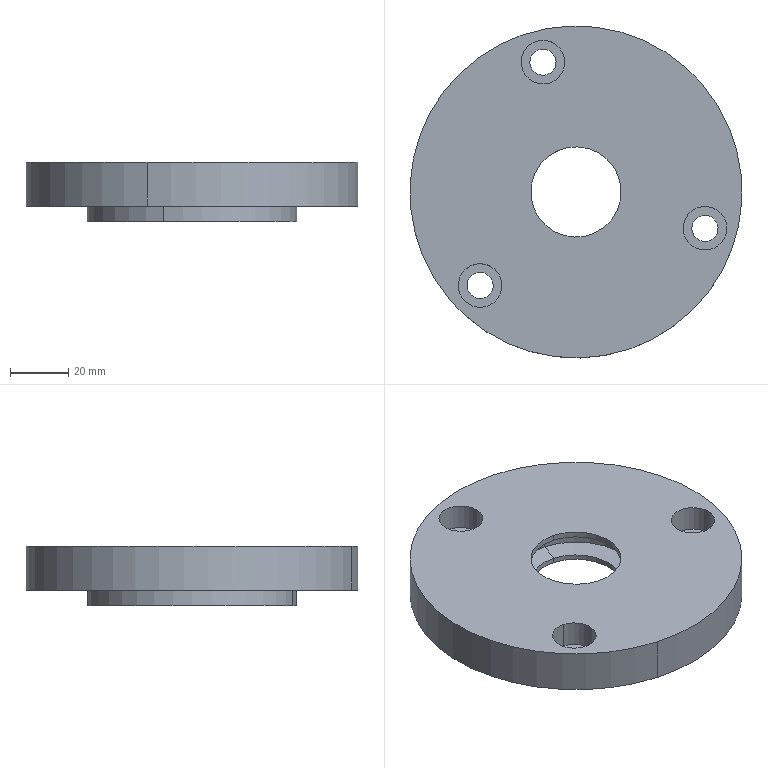Component | SolidWorks | 227-2 | 1 solid | 37 faces | box 114 x 114 x 20.3 mm | volume 130185 mm3 | cylinder 24 | plane 7 | cone 4 | torus 2 | commonest cylinder face diameters 15 x6 9 x6 31 x4 44 x2 60 x2 72 x2 114 x2
STEP:
#1=COLOUR_RGB('',0.7922,0.8196,0.9333);
#2=FILL_AREA_STYLE_COLOUR('',#1);
#3=FILL_AREA_STYLE('',(#2));
#4=SURFACE_STYLE_FILL_AREA(#3);
#5=SURFACE_SIDE_STYLE('',(#4));
#6=SURFACE_STYLE_USAGE(.BOTH.,#5);
#7=PRESENTATION_STYLE_ASSIGNMENT((#6));
#8=CARTESIAN_POINT('',(3.044,-0.8272,3.035));
#9=VERTEX_POINT('',#8);
#10=CARTESIAN_POINT('',(2.468,-2.874,3.035));
#11=VERTEX_POINT('',#10);
#12=CARTESIAN_POINT('',(2.756,-1.85,3.035));
#13=DIRECTION('',(0.,-0.,-1.));
#14=DIRECTION('',(-0.271,-0.9626,0.));
#15=AXIS2_PLACEMENT_3D('',#12,#13,#14);
#16=CIRCLE('',#15,1.063);
#17=EDGE_CURVE('',#9,#11,#16,.T.);
#18=ORIENTED_EDGE('',*,*,#17,.F.);
#19=CARTESIAN_POINT('',(3.076,-0.7135,2.917));
#20=VERTEX_POINT('',#19);
#21=CARTESIAN_POINT('',(3.044,-0.8272,2.917));
#22=DIRECTION('',(-0.9626,0.271,-0.));
#23=DIRECTION('',(-0.271,-0.9626,0.));
#24=AXIS2_PLACEMENT_3D('',#21,#22,#23);
#25=CIRCLE('',#24,0.1181);
#26=EDGE_CURVE('',#9,#20,#25,.T.);
#27=ORIENTED_EDGE('',*,*,#26,.T.);
#28=CARTESIAN_POINT('',(2.436,-2.987,2.917));
#29=VERTEX_POINT('',#28);
#30=CARTESIAN_POINT('',(2.756,-1.85,2.917));
#31=DIRECTION('',(-0.,0.,1.));
#32=DIRECTION('',(-0.271,-0.9626,0.));
#33=AXIS2_PLACEMENT_3D('',#30,#31,#32);
#34=CIRCLE('',#33,1.181);
#35=EDGE_CURVE('',#29,#20,#34,.T.);
#36=ORIENTED_EDGE('',*,*,#35,.F.);
#37=CARTESIAN_POINT('',(2.468,-2.874,2.917));
#38=DIRECTION('',(0.9626,-0.271,0.));
#39=DIRECTION('',(0.271,0.9626,0.));
#40=AXIS2_PLACEMENT_3D('',#37,#38,#39);
#41=CIRCLE('',#40,0.1181);
#42=EDGE_CURVE('',#11,#29,#41,.T.);
#43=ORIENTED_EDGE('',*,*,#42,.F.);
#44=EDGE_LOOP('',(#18,#27,#36,#43));
#45=FACE_OUTER_BOUND('',#44,.T.);
#46=CARTESIAN_POINT('',(2.756,-1.85,2.917));
#47=DIRECTION('',(0.,-0.,-1.));
#48=DIRECTION('',(-0.271,-0.9626,0.));
#49=AXIS2_PLACEMENT_3D('',#46,#47,#48);
#50=TOROIDAL_SURFACE('',#49,1.063,0.1181);
#51=ADVANCED_FACE('',(#45),#50,.F.);
#52=CARTESIAN_POINT('',(4.785,-2.268,3.13));
#53=VERTEX_POINT('',#52);
#54=CARTESIAN_POINT('',(4.213,-2.414,3.13));
#55=VERTEX_POINT('',#54);
#56=CARTESIAN_POINT('',(4.499,-2.341,3.13));
#57=DIRECTION('',(-0.,0.,1.));
#58=DIRECTION('',(-0.9691,-0.2466,0.));
#59=AXIS2_PLACEMENT_3D('',#56,#57,#58);
#60=CIRCLE('',#59,0.2953);
#61=EDGE_CURVE('',#53,#55,#60,.T.);
#62=ORIENTED_EDGE('',*,*,#61,.F.);
#63=CARTESIAN_POINT('',(4.785,-2.268,3.484));
#64=VERTEX_POINT('',#63);
#65=CARTESIAN_POINT('',(4.785,-2.268,3.13));
#66=DIRECTION('',(-0.,0.,1.));
#67=VECTOR('',#66,39.37);
#68=LINE('',#65,#67);
#69=EDGE_CURVE('',#53,#64,#68,.T.);
#70=ORIENTED_EDGE('',*,*,#69,.T.);
#71=CARTESIAN_POINT('',(4.213,-2.414,3.484));
#72=VERTEX_POINT('',#71);
#73=CARTESIAN_POINT('',(4.499,-2.341,3.484));
#74=DIRECTION('',(-0.,0.,1.));
#75=DIRECTION('',(-0.9691,-0.2466,0.));
#76=AXIS2_PLACEMENT_3D('',#73,#74,#75);
#77=CIRCLE('',#76,0.2953);
#78=EDGE_CURVE('',#64,#72,#77,.T.);
#79=ORIENTED_EDGE('',*,*,#78,.T.);
#80=CARTESIAN_POINT('',(4.213,-2.414,3.13));
#81=DIRECTION('',(-0.,0.,1.));
#82=VECTOR('',#81,39.37);
#83=LINE('',#80,#82);
#84=EDGE_CURVE('',#55,#72,#83,.T.);
#85=ORIENTED_EDGE('',*,*,#84,.F.);
#86=EDGE_LOOP('',(#62,#70,#79,#85));
#87=FACE_OUTER_BOUND('',#86,.T.);
#88=CARTESIAN_POINT('',(4.499,-2.341,3.13));
#89=DIRECTION('',(-0.,0.,1.));
#90=DIRECTION('',(-0.9691,-0.2466,0.));
#91=AXIS2_PLACEMENT_3D('',#88,#89,#90);
#92=CYLINDRICAL_SURFACE('',#91,0.2953);
#93=ADVANCED_FACE('',(#87),#92,.F.);
#94=CARTESIAN_POINT('',(2.103,0.1161,3.13));
#95=VERTEX_POINT('',#94);
#96=CARTESIAN_POINT('',(2.515,-0.3067,3.13));
#97=VERTEX_POINT('',#96);
#98=CARTESIAN_POINT('',(2.309,-0.09529,3.13));
#99=DIRECTION('',(-0.,0.,1.));
#100=DIRECTION('',(0.6981,-0.716,0.));
#101=AXIS2_PLACEMENT_3D('',#98,#99,#100);
#102=CIRCLE('',#101,0.2953);
#103=EDGE_CURVE('',#95,#97,#102,.T.);
#104=ORIENTED_EDGE('',*,*,#103,.F.);
#105=CARTESIAN_POINT('',(2.103,0.1161,3.484));
#106=VERTEX_POINT('',#105);
#107=CARTESIAN_POINT('',(2.103,0.1161,3.13));
#108=DIRECTION('',(-0.,0.,1.));
#109=VECTOR('',#108,39.37);
#110=LINE('',#107,#109);
#111=EDGE_CURVE('',#95,#106,#110,.T.);
#112=ORIENTED_EDGE('',*,*,#111,.T.);
#113=CARTESIAN_POINT('',(2.515,-0.3067,3.484));
#114=VERTEX_POINT('',#113);
#115=CARTESIAN_POINT('',(2.309,-0.09529,3.484));
#116=DIRECTION('',(-0.,0.,1.));
#117=DIRECTION('',(0.6981,-0.716,0.));
#118=AXIS2_PLACEMENT_3D('',#115,#116,#117);
#119=CIRCLE('',#118,0.2953);
#120=EDGE_CURVE('',#106,#114,#119,.T.);
#121=ORIENTED_EDGE('',*,*,#120,.T.);
#122=CARTESIAN_POINT('',(2.515,-0.3067,3.13));
#123=DIRECTION('',(-0.,0.,1.));
#124=VECTOR('',#123,39.37);
#125=LINE('',#122,#124);
#126=EDGE_CURVE('',#97,#114,#125,.T.);
#127=ORIENTED_EDGE('',*,*,#126,.F.);
#128=EDGE_LOOP('',(#104,#112,#121,#127));
#129=FACE_OUTER_BOUND('',#128,.T.);
#130=CARTESIAN_POINT('',(2.309,-0.09529,3.13));
#131=DIRECTION('',(-0.,0.,1.));
#132=DIRECTION('',(0.6981,-0.716,0.));
#133=AXIS2_PLACEMENT_3D('',#130,#131,#132);
#134=CYLINDRICAL_SURFACE('',#133,0.2953);
#135=ADVANCED_FACE('',(#129),#134,.F.);
#136=CARTESIAN_POINT('',(1.379,-3.399,3.13));
#137=VERTEX_POINT('',#136);
#138=CARTESIAN_POINT('',(1.539,-2.83,3.13));
#139=VERTEX_POINT('',#138);
#140=CARTESIAN_POINT('',(1.459,-3.115,3.13));
#141=DIRECTION('',(-0.,0.,1.));
#142=DIRECTION('',(0.271,0.9626,0.));
#143=AXIS2_PLACEMENT_3D('',#140,#141,#142);
#144=CIRCLE('',#143,0.2953);
#145=EDGE_CURVE('',#137,#139,#144,.T.);
#146=ORIENTED_EDGE('',*,*,#145,.F.);
#147=CARTESIAN_POINT('',(1.379,-3.399,3.484));
#148=VERTEX_POINT('',#147);
#149=CARTESIAN_POINT('',(1.379,-3.399,3.13));
#150=DIRECTION('',(-0.,0.,1.));
#151=VECTOR('',#150,39.37);
#152=LINE('',#149,#151);
#153=EDGE_CURVE('',#137,#148,#152,.T.);
#154=ORIENTED_EDGE('',*,*,#153,.T.);
#155=CARTESIAN_POINT('',(1.539,-2.83,3.484));
#156=VERTEX_POINT('',#155);
#157=CARTESIAN_POINT('',(1.459,-3.115,3.484));
#158=DIRECTION('',(-0.,0.,1.));
#159=DIRECTION('',(0.271,0.9626,0.));
#160=AXIS2_PLACEMENT_3D('',#157,#158,#159);
#161=CIRCLE('',#160,0.2953);
#162=EDGE_CURVE('',#148,#156,#161,.T.);
#163=ORIENTED_EDGE('',*,*,#162,.T.);
#164=CARTESIAN_POINT('',(1.539,-2.83,3.13));
#165=DIRECTION('',(-0.,0.,1.));
#166=VECTOR('',#165,39.37);
#167=LINE('',#164,#166);
#168=EDGE_CURVE('',#139,#156,#167,.T.);
#169=ORIENTED_EDGE('',*,*,#168,.F.);
#170=EDGE_LOOP('',(#146,#154,#163,#169));
#171=FACE_OUTER_BOUND('',#170,.T.);
#172=CARTESIAN_POINT('',(1.459,-3.115,3.13));
#173=DIRECTION('',(-0.,0.,1.));
#174=DIRECTION('',(0.271,0.9626,0.));
#175=AXIS2_PLACEMENT_3D('',#172,#173,#174);
#176=CYLINDRICAL_SURFACE('',#175,0.2953);
#177=ADVANCED_FACE('',(#171),#176,.F.);
#178=CARTESIAN_POINT('',(2.921,-1.263,3.106));
#179=VERTEX_POINT('',#178);
#180=CARTESIAN_POINT('',(2.591,-2.438,3.106));
#181=VERTEX_POINT('',#180);
#182=CARTESIAN_POINT('',(2.756,-1.85,3.106));
#183=DIRECTION('',(0.,-0.,-1.));
#184=DIRECTION('',(-0.271,-0.9626,0.));
#185=AXIS2_PLACEMENT_3D('',#182,#183,#184);
#186=CIRCLE('',#185,0.6102);
#187=EDGE_CURVE('',#179,#181,#186,.T.);
#188=ORIENTED_EDGE('',*,*,#187,.F.);
#189=CARTESIAN_POINT('',(2.921,-1.263,3.035));
#190=VERTEX_POINT('',#189);
#191=CARTESIAN_POINT('',(2.921,-1.263,2.783));
#192=DIRECTION('',(0.,-0.,-1.));
#193=VECTOR('',#192,39.37);
#194=LINE('',#191,#193);
#195=EDGE_CURVE('',#179,#190,#194,.T.);
#196=ORIENTED_EDGE('',*,*,#195,.T.);
#197=CARTESIAN_POINT('',(2.591,-2.438,3.035));
#198=VERTEX_POINT('',#197);
#199=CARTESIAN_POINT('',(2.756,-1.85,3.035));
#200=DIRECTION('',(0.,-0.,-1.));
#201=DIRECTION('',(-0.271,-0.9626,0.));
#202=AXIS2_PLACEMENT_3D('',#199,#200,#201);
#203=CIRCLE('',#202,0.6102);
#204=EDGE_CURVE('',#190,#198,#203,.T.);
#205=ORIENTED_EDGE('',*,*,#204,.T.);
#206=CARTESIAN_POINT('',(2.591,-2.438,2.783));
#207=DIRECTION('',(0.,-0.,-1.));
#208=VECTOR('',#207,39.37);
#209=LINE('',#206,#208);
#210=EDGE_CURVE('',#181,#198,#209,.T.);
#211=ORIENTED_EDGE('',*,*,#210,.F.);
#212=EDGE_LOOP('',(#188,#196,#205,#211));
#213=FACE_OUTER_BOUND('',#212,.T.);
#214=CARTESIAN_POINT('',(2.756,-1.85,2.783));
#215=DIRECTION('',(0.,-0.,-1.));
#216=DIRECTION('',(-0.271,-0.9626,0.));
#217=AXIS2_PLACEMENT_3D('',#214,#215,#216);
#218=CYLINDRICAL_SURFACE('',#217,0.6102);
#219=ADVANCED_FACE('',(#213),#218,.F.);
#220=ORIENTED_EDGE('',*,*,#187,.T.);
#221=CARTESIAN_POINT('',(2.521,-2.684,3.138));
#222=VERTEX_POINT('',#221);
#223=CARTESIAN_POINT('',(2.591,-2.438,3.106));
#224=DIRECTION('',(-0.269,-0.9554,0.1219));
#225=VECTOR('',#224,39.37);
#226=LINE('',#223,#225);
#227=EDGE_CURVE('',#181,#222,#226,.T.);
#228=ORIENTED_EDGE('',*,*,#227,.T.);
#229=CARTESIAN_POINT('',(2.991,-1.017,3.138));
#230=VERTEX_POINT('',#229);
#231=CARTESIAN_POINT('',(2.756,-1.85,3.138));
#232=DIRECTION('',(0.,-0.,-1.));
#233=DIRECTION('',(-0.271,-0.9626,0.));
#234=AXIS2_PLACEMENT_3D('',#231,#232,#233);
#235=CIRCLE('',#234,0.8661);
#236=EDGE_CURVE('',#230,#222,#235,.T.);
#237=ORIENTED_EDGE('',*,*,#236,.F.);
#238=CARTESIAN_POINT('',(2.921,-1.263,3.106));
#239=DIRECTION('',(0.269,0.9554,0.1219));
#240=VECTOR('',#239,39.37);
#241=LINE('',#238,#240);
#242=EDGE_CURVE('',#179,#230,#241,.T.);
#243=ORIENTED_EDGE('',*,*,#242,.F.);
#244=EDGE_LOOP('',(#220,#228,#237,#243));
#245=FACE_OUTER_BOUND('',#244,.T.);
#246=CARTESIAN_POINT('',(2.756,-1.85,3.106));
#247=DIRECTION('',(-0.,0.,1.));
#248=DIRECTION('',(0.271,0.9626,0.));
#249=AXIS2_PLACEMENT_3D('',#246,#247,#248);
#250=CONICAL_SURFACE('',#249,0.6102,1.449);
#251=ADVANCED_FACE('',(#245),#250,.F.);
#252=CARTESIAN_POINT('',(2.991,-1.017,3.374));
#253=VERTEX_POINT('',#252);
#254=CARTESIAN_POINT('',(2.521,-2.684,3.374));
#255=VERTEX_POINT('',#254);
#256=CARTESIAN_POINT('',(2.756,-1.85,3.374));
#257=DIRECTION('',(0.,-0.,-1.));
#258=DIRECTION('',(-0.271,-0.9626,0.));
#259=AXIS2_PLACEMENT_3D('',#256,#257,#258);
#260=CIRCLE('',#259,0.8661);
#261=EDGE_CURVE('',#253,#255,#260,.T.);
#262=ORIENTED_EDGE('',*,*,#261,.F.);
#263=CARTESIAN_POINT('',(2.991,-1.017,2.783));
#264=DIRECTION('',(0.,-0.,-1.));
#265=VECTOR('',#264,39.37);
#266=LINE('',#263,#265);
#267=EDGE_CURVE('',#253,#230,#266,.T.);
#268=ORIENTED_EDGE('',*,*,#267,.T.);
#269=ORIENTED_EDGE('',*,*,#236,.T.);
#270=CARTESIAN_POINT('',(2.521,-2.684,2.783));
#271=DIRECTION('',(0.,-0.,-1.));
#272=VECTOR('',#271,39.37);
#273=LINE('',#270,#272);
#274=EDGE_CURVE('',#255,#222,#273,.T.);
#275=ORIENTED_EDGE('',*,*,#274,.F.);
#276=EDGE_LOOP('',(#262,#268,#269,#275));
#277=FACE_OUTER_BOUND('',#276,.T.);
#278=CARTESIAN_POINT('',(2.756,-1.85,2.783));
#279=DIRECTION('',(0.,-0.,-1.));
#280=DIRECTION('',(-0.271,-0.9626,0.));
#281=AXIS2_PLACEMENT_3D('',#278,#279,#280);
#282=CYLINDRICAL_SURFACE('',#281,0.8661);
#283=ADVANCED_FACE('',(#277),#282,.F.);
#284=CARTESIAN_POINT('',(2.921,-1.263,3.405));
#285=VERTEX_POINT('',#284);
#286=CARTESIAN_POINT('',(2.591,-2.438,3.405));
#287=VERTEX_POINT('',#286);
#288=CARTESIAN_POINT('',(2.756,-1.85,3.405));
#289=DIRECTION('',(0.,-0.,-1.));
#290=DIRECTION('',(-0.271,-0.9626,0.));
#291=AXIS2_PLACEMENT_3D('',#288,#289,#290);
#292=CIRCLE('',#291,0.6102);
#293=EDGE_CURVE('',#285,#287,#292,.T.);
#294=ORIENTED_EDGE('',*,*,#293,.F.);
#295=CARTESIAN_POINT('',(2.991,-1.017,3.374));
#296=DIRECTION('',(0.269,0.9554,-0.1219));
#297=VECTOR('',#296,39.37);
#298=LINE('',#295,#297);
#299=EDGE_CURVE('',#285,#253,#298,.T.);
#300=ORIENTED_EDGE('',*,*,#299,.T.);
#301=ORIENTED_EDGE('',*,*,#261,.T.);
#302=CARTESIAN_POINT('',(2.521,-2.684,3.374));
#303=DIRECTION('',(-0.269,-0.9554,-0.1219));
#304=VECTOR('',#303,39.37);
#305=LINE('',#302,#304);
#306=EDGE_CURVE('',#287,#255,#305,.T.);
#307=ORIENTED_EDGE('',*,*,#306,.F.);
#308=EDGE_LOOP('',(#294,#300,#301,#307));
#309=FACE_OUTER_BOUND('',#308,.T.);
#310=CARTESIAN_POINT('',(2.756,-1.85,3.374));
#311=DIRECTION('',(0.,-0.,-1.));
#312=DIRECTION('',(-0.271,-0.9626,0.));
#313=AXIS2_PLACEMENT_3D('',#310,#311,#312);
#314=CONICAL_SURFACE('',#313,0.8661,1.449);
#315=ADVANCED_FACE('',(#309),#314,.F.);
#316=CARTESIAN_POINT('',(2.921,-1.263,3.484));
#317=VERTEX_POINT('',#316);
#318=CARTESIAN_POINT('',(2.591,-2.438,3.484));
#319=VERTEX_POINT('',#318);
#320=CARTESIAN_POINT('',(2.756,-1.85,3.484));
#321=DIRECTION('',(0.,-0.,-1.));
#322=DIRECTION('',(-0.271,-0.9626,0.));
#323=AXIS2_PLACEMENT_3D('',#320,#321,#322);
#324=CIRCLE('',#323,0.6102);
#325=EDGE_CURVE('',#317,#319,#324,.T.);
#326=ORIENTED_EDGE('',*,*,#325,.F.);
#327=CARTESIAN_POINT('',(2.921,-1.263,2.783));
#328=DIRECTION('',(0.,-0.,-1.));
#329=VECTOR('',#328,39.37);
#330=LINE('',#327,#329);
#331=EDGE_CURVE('',#317,#285,#330,.T.);
#332=ORIENTED_EDGE('',*,*,#331,.T.);
#333=ORIENTED_EDGE('',*,*,#293,.T.);
#334=CARTESIAN_POINT('',(2.591,-2.438,2.783));
#335=DIRECTION('',(0.,-0.,-1.));
#336=VECTOR('',#335,39.37);
#337=LINE('',#334,#336);
#338=EDGE_CURVE('',#319,#287,#337,.T.);
#339=ORIENTED_EDGE('',*,*,#338,.F.);
#340=EDGE_LOOP('',(#326,#332,#333,#339));
#341=FACE_OUTER_BOUND('',#340,.T.);
#342=CARTESIAN_POINT('',(2.756,-1.85,2.783));
#343=DIRECTION('',(0.,-0.,-1.));
#344=DIRECTION('',(-0.271,-0.9626,0.));
#345=AXIS2_PLACEMENT_3D('',#342,#343,#344);
#346=CYLINDRICAL_SURFACE('',#345,0.6102);
#347=ADVANCED_FACE('',(#341),#346,.F.);
#348=ORIENTED_EDGE('',*,*,#35,.T.);
#349=CARTESIAN_POINT('',(3.076,-0.7135,2.685));
#350=VERTEX_POINT('',#349);
#351=CARTESIAN_POINT('',(3.076,-0.7135,6.825));
#352=DIRECTION('',(0.,-0.,-1.));
#353=VECTOR('',#352,39.37);
#354=LINE('',#351,#353);
#355=EDGE_CURVE('',#20,#350,#354,.T.);
#356=ORIENTED_EDGE('',*,*,#355,.T.);
#357=CARTESIAN_POINT('',(2.436,-2.987,2.685));
#358=VERTEX_POINT('',#357);
#359=CARTESIAN_POINT('',(2.756,-1.85,2.685));
#360=DIRECTION('',(0.,-0.,-1.));
#361=DIRECTION('',(-0.271,-0.9626,0.));
#362=AXIS2_PLACEMENT_3D('',#359,#360,#361);
#363=CIRCLE('',#362,1.181);
#364=EDGE_CURVE('',#350,#358,#363,.T.);
#365=ORIENTED_EDGE('',*,*,#364,.T.);
#366=CARTESIAN_POINT('',(2.436,-2.987,6.825));
#367=DIRECTION('',(0.,-0.,-1.));
#368=VECTOR('',#367,39.37);
#369=LINE('',#366,#368);
#370=EDGE_CURVE('',#29,#358,#369,.T.);
#371=ORIENTED_EDGE('',*,*,#370,.F.);
#372=EDGE_LOOP('',(#348,#356,#365,#371));
#373=FACE_OUTER_BOUND('',#372,.T.);
#374=CARTESIAN_POINT('',(2.756,-1.85,6.825));
#375=DIRECTION('',(0.,-0.,-1.));
#376=DIRECTION('',(-0.271,-0.9626,0.));
#377=AXIS2_PLACEMENT_3D('',#374,#375,#376);
#378=CYLINDRICAL_SURFACE('',#377,1.181);
#379=ADVANCED_FACE('',(#373),#378,.F.);
#380=CARTESIAN_POINT('',(2.372,-3.215,2.685));
#381=VERTEX_POINT('',#380);
#382=CARTESIAN_POINT('',(3.14,-0.4861,2.685));
#383=VERTEX_POINT('',#382);
#384=CARTESIAN_POINT('',(2.756,-1.85,2.685));
#385=DIRECTION('',(0.,-0.,-1.));
#386=DIRECTION('',(-0.271,-0.9626,0.));
#387=AXIS2_PLACEMENT_3D('',#384,#385,#386);
#388=CIRCLE('',#387,1.417);
#389=EDGE_CURVE('',#381,#383,#388,.T.);
#390=ORIENTED_EDGE('',*,*,#389,.F.);
#391=CARTESIAN_POINT('',(2.372,-3.215,2.894));
#392=VERTEX_POINT('',#391);
#393=CARTESIAN_POINT('',(2.372,-3.215,2.685));
#394=DIRECTION('',(-0.,0.,1.));
#395=VECTOR('',#394,39.37);
#396=LINE('',#393,#395);
#397=EDGE_CURVE('',#381,#392,#396,.T.);
#398=ORIENTED_EDGE('',*,*,#397,.T.);
#399=CARTESIAN_POINT('',(3.14,-0.4861,2.894));
#400=VERTEX_POINT('',#399);
#401=CARTESIAN_POINT('',(2.756,-1.85,2.894));
#402=DIRECTION('',(0.,-0.,-1.));
#403=DIRECTION('',(-0.271,-0.9626,0.));
#404=AXIS2_PLACEMENT_3D('',#401,#402,#403);
#405=CIRCLE('',#404,1.417);
#406=EDGE_CURVE('',#392,#400,#405,.T.);
#407=ORIENTED_EDGE('',*,*,#406,.T.);
#408=CARTESIAN_POINT('',(3.14,-0.4861,2.685));
#409=DIRECTION('',(-0.,0.,1.));
#410=VECTOR('',#409,39.37);
#411=LINE('',#408,#410);
#412=EDGE_CURVE('',#383,#400,#411,.T.);
#413=ORIENTED_EDGE('',*,*,#412,.F.);
#414=EDGE_LOOP('',(#390,#398,#407,#413));
#415=FACE_OUTER_BOUND('',#414,.T.);
#416=CARTESIAN_POINT('',(2.756,-1.85,2.685));
#417=DIRECTION('',(-0.,0.,1.));
#418=DIRECTION('',(0.271,0.9626,0.));
#419=AXIS2_PLACEMENT_3D('',#416,#417,#418);
#420=CYLINDRICAL_SURFACE('',#419,1.417);
#421=ADVANCED_FACE('',(#415),#420,.T.);
#422=CARTESIAN_POINT('',(2.148,-4.011,2.894));
#423=VERTEX_POINT('',#422);
#424=CARTESIAN_POINT('',(3.364,0.3097,2.894));
#425=VERTEX_POINT('',#424);
#426=CARTESIAN_POINT('',(2.756,-1.85,2.894));
#427=DIRECTION('',(0.,-0.,-1.));
#428=DIRECTION('',(-0.271,-0.9626,0.));
#429=AXIS2_PLACEMENT_3D('',#426,#427,#428);
#430=CIRCLE('',#429,2.244);
#431=EDGE_CURVE('',#423,#425,#430,.T.);
#432=ORIENTED_EDGE('',*,*,#431,.F.);
#433=CARTESIAN_POINT('',(2.148,-4.011,3.484));
#434=VERTEX_POINT('',#433);
#435=CARTESIAN_POINT('',(2.148,-4.011,2.894));
#436=DIRECTION('',(-0.,0.,1.));
#437=VECTOR('',#436,39.37);
#438=LINE('',#435,#437);
#439=EDGE_CURVE('',#423,#434,#438,.T.);
#440=ORIENTED_EDGE('',*,*,#439,.T.);
#441=CARTESIAN_POINT('',(3.364,0.3097,3.484));
#442=VERTEX_POINT('',#441);
#443=CARTESIAN_POINT('',(2.756,-1.85,3.484));
#444=DIRECTION('',(0.,-0.,-1.));
#445=DIRECTION('',(-0.271,-0.9626,0.));
#446=AXIS2_PLACEMENT_3D('',#443,#444,#445);
#447=CIRCLE('',#446,2.244);
#448=EDGE_CURVE('',#434,#442,#447,.T.);
#449=ORIENTED_EDGE('',*,*,#448,.T.);
#450=CARTESIAN_POINT('',(3.364,0.3097,2.894));
#451=DIRECTION('',(-0.,0.,1.));
#452=VECTOR('',#451,39.37);
#453=LINE('',#450,#452);
#454=EDGE_CURVE('',#425,#442,#453,.T.);
#455=ORIENTED_EDGE('',*,*,#454,.F.);
#456=EDGE_LOOP('',(#432,#440,#449,#455));
#457=FACE_OUTER_BOUND('',#456,.T.);
#458=CARTESIAN_POINT('',(2.756,-1.85,2.894));
#459=DIRECTION('',(-0.,0.,1.));
#460=DIRECTION('',(0.271,0.9626,0.));
#461=AXIS2_PLACEMENT_3D('',#458,#459,#460);
#462=CYLINDRICAL_SURFACE('',#461,2.244);
#463=ADVANCED_FACE('',(#457),#462,.T.);
#464=CARTESIAN_POINT('',(1.507,-2.944,2.894));
#465=VERTEX_POINT('',#464);
#466=CARTESIAN_POINT('',(1.411,-3.285,2.894));
#467=VERTEX_POINT('',#466);
#468=CARTESIAN_POINT('',(1.459,-3.115,2.894));
#469=DIRECTION('',(0.,-0.,-1.));
#470=DIRECTION('',(-0.271,-0.9626,0.));
#471=AXIS2_PLACEMENT_3D('',#468,#469,#470);
#472=CIRCLE('',#471,0.1772);
#473=EDGE_CURVE('',#465,#467,#472,.T.);
#474=ORIENTED_EDGE('',*,*,#473,.T.);
#475=CARTESIAN_POINT('',(1.411,-3.285,3.13));
#476=VERTEX_POINT('',#475);
#477=CARTESIAN_POINT('',(1.411,-3.285,2.894));
#478=DIRECTION('',(-0.,0.,1.));
#479=VECTOR('',#478,39.37);
#480=LINE('',#477,#479);
#481=EDGE_CURVE('',#467,#476,#480,.T.);
#482=ORIENTED_EDGE('',*,*,#481,.T.);
#483=CARTESIAN_POINT('',(1.507,-2.944,3.13));
#484=VERTEX_POINT('',#483);
#485=CARTESIAN_POINT('',(1.459,-3.115,3.13));
#486=DIRECTION('',(-0.,0.,1.));
#487=DIRECTION('',(0.271,0.9626,0.));
#488=AXIS2_PLACEMENT_3D('',#485,#486,#487);
#489=CIRCLE('',#488,0.1772);
#490=EDGE_CURVE('',#476,#484,#489,.T.);
#491=ORIENTED_EDGE('',*,*,#490,.T.);
#492=CARTESIAN_POINT('',(1.507,-2.944,2.894));
#493=DIRECTION('',(-0.,0.,1.));
#494=VECTOR('',#493,39.37);
#495=LINE('',#492,#494);
#496=EDGE_CURVE('',#465,#484,#495,.T.);
#497=ORIENTED_EDGE('',*,*,#496,.F.);
#498=EDGE_LOOP('',(#474,#482,#491,#497));
#499=FACE_OUTER_BOUND('',#498,.T.);
#500=CARTESIAN_POINT('',(1.459,-3.115,2.894));
#501=DIRECTION('',(-0.,0.,1.));
#502=DIRECTION('',(0.271,0.9626,0.));
#503=AXIS2_PLACEMENT_3D('',#500,#501,#502);
#504=CYLINDRICAL_SURFACE('',#503,0.1772);
#505=ADVANCED_FACE('',(#499),#504,.F.);
#506=CARTESIAN_POINT('',(2.357,0.07525,2.894));
#507=VERTEX_POINT('',#506);
#508=CARTESIAN_POINT('',(2.261,-0.2658,2.894));
#509=VERTEX_POINT('',#508);
#510=CARTESIAN_POINT('',(2.309,-0.09529,2.894));
#511=DIRECTION('',(0.,-0.,-1.));
#512=DIRECTION('',(-0.271,-0.9626,0.));
#513=AXIS2_PLACEMENT_3D('',#510,#511,#512);
#514=CIRCLE('',#513,0.1772);
#515=EDGE_CURVE('',#507,#509,#514,.T.);
#516=ORIENTED_EDGE('',*,*,#515,.T.);
#517=CARTESIAN_POINT('',(2.261,-0.2658,3.13));
#518=VERTEX_POINT('',#517);
#519=CARTESIAN_POINT('',(2.261,-0.2658,2.894));
#520=DIRECTION('',(-0.,0.,1.));
#521=VECTOR('',#520,39.37);
#522=LINE('',#519,#521);
#523=EDGE_CURVE('',#509,#518,#522,.T.);
#524=ORIENTED_EDGE('',*,*,#523,.T.);
#525=CARTESIAN_POINT('',(2.357,0.07525,3.13));
#526=VERTEX_POINT('',#525);
#527=CARTESIAN_POINT('',(2.309,-0.09529,3.13));
#528=DIRECTION('',(-0.,0.,1.));
#529=DIRECTION('',(0.271,0.9626,0.));
#530=AXIS2_PLACEMENT_3D('',#527,#528,#529);
#531=CIRCLE('',#530,0.1772);
#532=EDGE_CURVE('',#518,#526,#531,.T.);
#533=ORIENTED_EDGE('',*,*,#532,.T.);
#534=CARTESIAN_POINT('',(2.357,0.07525,2.894));
#535=DIRECTION('',(-0.,0.,1.));
#536=VECTOR('',#535,39.37);
#537=LINE('',#534,#536);
#538=EDGE_CURVE('',#507,#526,#537,.T.);
#539=ORIENTED_EDGE('',*,*,#538,.F.);
#540=EDGE_LOOP('',(#516,#524,#533,#539));
#541=FACE_OUTER_BOUND('',#540,.T.);
#542=CARTESIAN_POINT('',(2.309,-0.09529,2.894));
#543=DIRECTION('',(-0.,0.,1.));
#544=DIRECTION('',(0.271,0.9626,0.));
#545=AXIS2_PLACEMENT_3D('',#542,#543,#544);
#546=CYLINDRICAL_SURFACE('',#545,0.1772);
#547=ADVANCED_FACE('',(#541),#546,.F.);
#548=CARTESIAN_POINT('',(4.547,-2.171,2.894));
#549=VERTEX_POINT('',#548);
#550=CARTESIAN_POINT('',(4.451,-2.512,2.894));
#551=VERTEX_POINT('',#550);
#552=CARTESIAN_POINT('',(4.499,-2.341,2.894));
#553=DIRECTION('',(0.,-0.,-1.));
#554=DIRECTION('',(-0.271,-0.9626,0.));
#555=AXIS2_PLACEMENT_3D('',#552,#553,#554);
#556=CIRCLE('',#555,0.1772);
#557=EDGE_CURVE('',#549,#551,#556,.T.);
#558=ORIENTED_EDGE('',*,*,#557,.T.);
#559=CARTESIAN_POINT('',(4.451,-2.512,3.13));
#560=VERTEX_POINT('',#559);
#561=CARTESIAN_POINT('',(4.451,-2.512,2.894));
#562=DIRECTION('',(-0.,0.,1.));
#563=VECTOR('',#562,39.37);
#564=LINE('',#561,#563);
#565=EDGE_CURVE('',#551,#560,#564,.T.);
#566=ORIENTED_EDGE('',*,*,#565,.T.);
#567=CARTESIAN_POINT('',(4.547,-2.171,3.13));
#568=VERTEX_POINT('',#567);
#569=CARTESIAN_POINT('',(4.499,-2.341,3.13));
#570=DIRECTION('',(-0.,0.,1.));
#571=DIRECTION('',(0.271,0.9626,0.));
#572=AXIS2_PLACEMENT_3D('',#569,#570,#571);
#573=CIRCLE('',#572,0.1772);
#574=EDGE_CURVE('',#560,#568,#573,.T.);
#575=ORIENTED_EDGE('',*,*,#574,.T.);
#576=CARTESIAN_POINT('',(4.547,-2.171,2.894));
#577=DIRECTION('',(-0.,0.,1.));
#578=VECTOR('',#577,39.37);
#579=LINE('',#576,#578);
#580=EDGE_CURVE('',#549,#568,#579,.T.);
#581=ORIENTED_EDGE('',*,*,#580,.F.);
#582=EDGE_LOOP('',(#558,#566,#575,#581));
#583=FACE_OUTER_BOUND('',#582,.T.);
#584=CARTESIAN_POINT('',(4.499,-2.341,2.894));
#585=DIRECTION('',(-0.,0.,1.));
#586=DIRECTION('',(0.271,0.9626,0.));
#587=AXIS2_PLACEMENT_3D('',#584,#585,#586);
#588=CYLINDRICAL_SURFACE('',#587,0.1772);
#589=ADVANCED_FACE('',(#583),#588,.F.);
#590=ORIENTED_EDGE('',*,*,#565,.F.);
#591=CARTESIAN_POINT('',(4.499,-2.341,2.894));
#592=DIRECTION('',(0.,-0.,-1.));
#593=DIRECTION('',(-0.271,-0.9626,0.));
#594=AXIS2_PLACEMENT_3D('',#591,#592,#593);
#595=CIRCLE('',#594,0.1772);
#596=EDGE_CURVE('',#551,#549,#595,.T.);
#597=ORIENTED_EDGE('',*,*,#596,.T.);
#598=ORIENTED_EDGE('',*,*,#580,.T.);
#599=CARTESIAN_POINT('',(4.499,-2.341,3.13));
#600=DIRECTION('',(-0.,0.,1.));
#601=DIRECTION('',(0.271,0.9626,0.));
#602=AXIS2_PLACEMENT_3D('',#599,#600,#601);
#603=CIRCLE('',#602,0.1772);
#604=EDGE_CURVE('',#568,#560,#603,.T.);
#605=ORIENTED_EDGE('',*,*,#604,.T.);
#606=EDGE_LOOP('',(#590,#597,#598,#605));
#607=FACE_OUTER_BOUND('',#606,.T.);
#608=CARTESIAN_POINT('',(4.499,-2.341,2.894));
#609=DIRECTION('',(-0.,0.,1.));
#610=DIRECTION('',(0.271,0.9626,0.));
#611=AXIS2_PLACEMENT_3D('',#608,#609,#610);
#612=CYLINDRICAL_SURFACE('',#611,0.1772);
#613=ADVANCED_FACE('',(#607),#612,.F.);
#614=ORIENTED_EDGE('',*,*,#523,.F.);
#615=CARTESIAN_POINT('',(2.309,-0.09529,2.894));
#616=DIRECTION('',(0.,-0.,-1.));
#617=DIRECTION('',(-0.271,-0.9626,0.));
#618=AXIS2_PLACEMENT_3D('',#615,#616,#617);
#619=CIRCLE('',#618,0.1772);
#620=EDGE_CURVE('',#509,#507,#619,.T.);
#621=ORIENTED_EDGE('',*,*,#620,.T.);
#622=ORIENTED_EDGE('',*,*,#538,.T.);
#623=CARTESIAN_POINT('',(2.309,-0.09529,3.13));
#624=DIRECTION('',(-0.,0.,1.));
#625=DIRECTION('',(0.271,0.9626,0.));
#626=AXIS2_PLACEMENT_3D('',#623,#624,#625);
#627=CIRCLE('',#626,0.1772);
#628=EDGE_CURVE('',#526,#518,#627,.T.);
#629=ORIENTED_EDGE('',*,*,#628,.T.);
#630=EDGE_LOOP('',(#614,#621,#622,#629));
#631=FACE_OUTER_BOUND('',#630,.T.);
#632=CARTESIAN_POINT('',(2.309,-0.09529,2.894));
#633=DIRECTION('',(-0.,0.,1.));
#634=DIRECTION('',(0.271,0.9626,0.));
#635=AXIS2_PLACEMENT_3D('',#632,#633,#634);
#636=CYLINDRICAL_SURFACE('',#635,0.1772);
#637=ADVANCED_FACE('',(#631),#636,.F.);
#638=ORIENTED_EDGE('',*,*,#481,.F.);
#639=CARTESIAN_POINT('',(1.459,-3.115,2.894));
#640=DIRECTION('',(0.,-0.,-1.));
#641=DIRECTION('',(-0.271,-0.9626,0.));
#642=AXIS2_PLACEMENT_3D('',#639,#640,#641);
#643=CIRCLE('',#642,0.1772);
#644=EDGE_CURVE('',#467,#465,#643,.T.);
#645=ORIENTED_EDGE('',*,*,#644,.T.);
#646=ORIENTED_EDGE('',*,*,#496,.T.);
#647=CARTESIAN_POINT('',(1.459,-3.115,3.13));
#648=DIRECTION('',(-0.,0.,1.));
#649=DIRECTION('',(0.271,0.9626,0.));
#650=AXIS2_PLACEMENT_3D('',#647,#648,#649);
#651=CIRCLE('',#650,0.1772);
#652=EDGE_CURVE('',#484,#476,#651,.T.);
#653=ORIENTED_EDGE('',*,*,#652,.T.);
#654=EDGE_LOOP('',(#638,#645,#646,#653));
#655=FACE_OUTER_BOUND('',#654,.T.);
#656=CARTESIAN_POINT('',(1.459,-3.115,2.894));
#657=DIRECTION('',(-0.,0.,1.));
#658=DIRECTION('',(0.271,0.9626,0.));
#659=AXIS2_PLACEMENT_3D('',#656,#657,#658);
#660=CYLINDRICAL_SURFACE('',#659,0.1772);
#661=ADVANCED_FACE('',(#655),#660,.F.);
#662=CARTESIAN_POINT('',(2.756,-1.85,2.894));
#663=DIRECTION('',(0.,-0.,-1.));
#664=DIRECTION('',(-0.271,-0.9626,0.));
#665=AXIS2_PLACEMENT_3D('',#662,#663,#664);
#666=CIRCLE('',#665,1.417);
#667=EDGE_CURVE('',#400,#392,#666,.T.);
#668=ORIENTED_EDGE('',*,*,#667,.F.);
#669=ORIENTED_EDGE('',*,*,#406,.F.);
#670=EDGE_LOOP('',(#668,#669));
#671=FACE_BOUND('',#670,.T.);
#672=ORIENTED_EDGE('',*,*,#515,.F.);
#673=ORIENTED_EDGE('',*,*,#620,.F.);
#674=EDGE_LOOP('',(#672,#673));
#675=FACE_BOUND('',#674,.T.);
#676=CARTESIAN_POINT('',(2.756,-1.85,2.894));
#677=DIRECTION('',(0.,-0.,-1.));
#678=DIRECTION('',(-0.271,-0.9626,0.));
#679=AXIS2_PLACEMENT_3D('',#676,#677,#678);
#680=CIRCLE('',#679,2.244);
#681=EDGE_CURVE('',#425,#423,#680,.T.);
#682=ORIENTED_EDGE('',*,*,#681,.T.);
#683=ORIENTED_EDGE('',*,*,#431,.T.);
#684=EDGE_LOOP('',(#682,#683));
#685=FACE_OUTER_BOUND('',#684,.T.);
#686=ORIENTED_EDGE('',*,*,#557,.F.);
#687=ORIENTED_EDGE('',*,*,#596,.F.);
#688=EDGE_LOOP('',(#686,#687));
#689=FACE_BOUND('',#688,.T.);
#690=ORIENTED_EDGE('',*,*,#473,.F.);
#691=ORIENTED_EDGE('',*,*,#644,.F.);
#692=EDGE_LOOP('',(#690,#691));
#693=FACE_BOUND('',#692,.T.);
#694=CARTESIAN_POINT('',(2.756,-1.85,2.894));
#695=DIRECTION('',(0.,-0.,-1.));
#696=DIRECTION('',(-0.271,-0.9626,0.));
#697=AXIS2_PLACEMENT_3D('',#694,#695,#696);
#698=PLANE('',#697);
#699=ADVANCED_FACE('',(#671,#675,#685,#689,#693),#698,.T.);
#700=CARTESIAN_POINT('',(2.309,-0.09529,3.484));
#701=DIRECTION('',(-0.,0.,1.));
#702=DIRECTION('',(0.6981,-0.716,0.));
#703=AXIS2_PLACEMENT_3D('',#700,#701,#702);
#704=CIRCLE('',#703,0.2953);
#705=EDGE_CURVE('',#114,#106,#704,.T.);
#706=ORIENTED_EDGE('',*,*,#705,.F.);
#707=ORIENTED_EDGE('',*,*,#120,.F.);
#708=EDGE_LOOP('',(#706,#707));
#709=FACE_BOUND('',#708,.T.);
#710=CARTESIAN_POINT('',(4.499,-2.341,3.484));
#711=DIRECTION('',(-0.,0.,1.));
#712=DIRECTION('',(-0.9691,-0.2466,0.));
#713=AXIS2_PLACEMENT_3D('',#710,#711,#712);
#714=CIRCLE('',#713,0.2953);
#715=EDGE_CURVE('',#72,#64,#714,.T.);
#716=ORIENTED_EDGE('',*,*,#715,.F.);
#717=ORIENTED_EDGE('',*,*,#78,.F.);
#718=EDGE_LOOP('',(#716,#717));
#719=FACE_BOUND('',#718,.T.);
#720=CARTESIAN_POINT('',(1.459,-3.115,3.484));
#721=DIRECTION('',(-0.,0.,1.));
#722=DIRECTION('',(0.271,0.9626,0.));
#723=AXIS2_PLACEMENT_3D('',#720,#721,#722);
#724=CIRCLE('',#723,0.2953);
#725=EDGE_CURVE('',#156,#148,#724,.T.);
#726=ORIENTED_EDGE('',*,*,#725,.F.);
#727=ORIENTED_EDGE('',*,*,#162,.F.);
#728=EDGE_LOOP('',(#726,#727));
#729=FACE_BOUND('',#728,.T.);
#730=CARTESIAN_POINT('',(2.756,-1.85,3.484));
#731=DIRECTION('',(0.,-0.,-1.));
#732=DIRECTION('',(-0.271,-0.9626,0.));
#733=AXIS2_PLACEMENT_3D('',#730,#731,#732);
#734=CIRCLE('',#733,0.6102);
#735=EDGE_CURVE('',#319,#317,#734,.T.);
#736=ORIENTED_EDGE('',*,*,#735,.T.);
#737=ORIENTED_EDGE('',*,*,#325,.T.);
#738=EDGE_LOOP('',(#736,#737));
#739=FACE_BOUND('',#738,.T.);
#740=CARTESIAN_POINT('',(2.756,-1.85,3.484));
#741=DIRECTION('',(0.,-0.,-1.));
#742=DIRECTION('',(-0.271,-0.9626,0.));
#743=AXIS2_PLACEMENT_3D('',#740,#741,#742);
#744=CIRCLE('',#743,2.244);
#745=EDGE_CURVE('',#442,#434,#744,.T.);
#746=ORIENTED_EDGE('',*,*,#745,.F.);
#747=ORIENTED_EDGE('',*,*,#448,.F.);
#748=EDGE_LOOP('',(#746,#747));
#749=FACE_OUTER_BOUND('',#748,.T.);
#750=CARTESIAN_POINT('',(2.756,-1.85,3.484));
#751=DIRECTION('',(0.,-0.,-1.));
#752=DIRECTION('',(-0.271,-0.9626,0.));
#753=AXIS2_PLACEMENT_3D('',#750,#751,#752);
#754=PLANE('',#753);
#755=ADVANCED_FACE('',(#709,#719,#729,#739,#749),#754,.F.);
#756=ORIENTED_EDGE('',*,*,#439,.F.);
#757=ORIENTED_EDGE('',*,*,#681,.F.);
#758=ORIENTED_EDGE('',*,*,#454,.T.);
#759=ORIENTED_EDGE('',*,*,#745,.T.);
#760=EDGE_LOOP('',(#756,#757,#758,#759));
#761=FACE_OUTER_BOUND('',#760,.T.);
#762=CARTESIAN_POINT('',(2.756,-1.85,2.894));
#763=DIRECTION('',(-0.,0.,1.));
#764=DIRECTION('',(0.271,0.9626,0.));
#765=AXIS2_PLACEMENT_3D('',#762,#763,#764);
#766=CYLINDRICAL_SURFACE('',#765,2.244);
#767=ADVANCED_FACE('',(#761),#766,.T.);
#768=ORIENTED_EDGE('',*,*,#397,.F.);
#769=CARTESIAN_POINT('',(2.756,-1.85,2.685));
#770=DIRECTION('',(0.,-0.,-1.));
#771=DIRECTION('',(-0.271,-0.9626,0.));
#772=AXIS2_PLACEMENT_3D('',#769,#770,#771);
#773=CIRCLE('',#772,1.417);
#774=EDGE_CURVE('',#383,#381,#773,.T.);
#775=ORIENTED_EDGE('',*,*,#774,.F.);
#776=ORIENTED_EDGE('',*,*,#412,.T.);
#777=ORIENTED_EDGE('',*,*,#667,.T.);
#778=EDGE_LOOP('',(#768,#775,#776,#777));
#779=FACE_OUTER_BOUND('',#778,.T.);
#780=CARTESIAN_POINT('',(2.756,-1.85,2.685));
#781=DIRECTION('',(-0.,0.,1.));
#782=DIRECTION('',(0.271,0.9626,0.));
#783=AXIS2_PLACEMENT_3D('',#780,#781,#782);
#784=CYLINDRICAL_SURFACE('',#783,1.417);
#785=ADVANCED_FACE('',(#779),#784,.T.);
#786=CARTESIAN_POINT('',(2.756,-1.85,2.685));
#787=DIRECTION('',(0.,-0.,-1.));
#788=DIRECTION('',(-0.271,-0.9626,0.));
#789=AXIS2_PLACEMENT_3D('',#786,#787,#788);
#790=CIRCLE('',#789,1.181);
#791=EDGE_CURVE('',#358,#350,#790,.T.);
#792=ORIENTED_EDGE('',*,*,#791,.F.);
#793=ORIENTED_EDGE('',*,*,#364,.F.);
#794=EDGE_LOOP('',(#792,#793));
#795=FACE_BOUND('',#794,.T.);
#796=ORIENTED_EDGE('',*,*,#774,.T.);
#797=ORIENTED_EDGE('',*,*,#389,.T.);
#798=EDGE_LOOP('',(#796,#797));
#799=FACE_OUTER_BOUND('',#798,.T.);
#800=CARTESIAN_POINT('',(2.756,-1.85,2.685));
#801=DIRECTION('',(0.,-0.,-1.));
#802=DIRECTION('',(-0.271,-0.9626,0.));
#803=AXIS2_PLACEMENT_3D('',#800,#801,#802);
#804=PLANE('',#803);
#805=ADVANCED_FACE('',(#795,#799),#804,.T.);
#806=ORIENTED_EDGE('',*,*,#355,.F.);
#807=CARTESIAN_POINT('',(2.756,-1.85,2.917));
#808=DIRECTION('',(-0.,0.,1.));
#809=DIRECTION('',(-0.271,-0.9626,0.));
#810=AXIS2_PLACEMENT_3D('',#807,#808,#809);
#811=CIRCLE('',#810,1.181);
#812=EDGE_CURVE('',#20,#29,#811,.T.);
#813=ORIENTED_EDGE('',*,*,#812,.T.);
#814=ORIENTED_EDGE('',*,*,#370,.T.);
#815=ORIENTED_EDGE('',*,*,#791,.T.);
#816=EDGE_LOOP('',(#806,#813,#814,#815));
#817=FACE_OUTER_BOUND('',#816,.T.);
#818=CARTESIAN_POINT('',(2.756,-1.85,6.825));
#819=DIRECTION('',(0.,-0.,-1.));
#820=DIRECTION('',(-0.271,-0.9626,0.));
#821=AXIS2_PLACEMENT_3D('',#818,#819,#820);
#822=CYLINDRICAL_SURFACE('',#821,1.181);
#823=ADVANCED_FACE('',(#817),#822,.F.);
#824=CARTESIAN_POINT('',(2.756,-1.85,3.035));
#825=DIRECTION('',(0.,-0.,-1.));
#826=DIRECTION('',(-0.271,-0.9626,0.));
#827=AXIS2_PLACEMENT_3D('',#824,#825,#826);
#828=CIRCLE('',#827,1.063);
#829=EDGE_CURVE('',#11,#9,#828,.T.);
#830=ORIENTED_EDGE('',*,*,#829,.T.);
#831=ORIENTED_EDGE('',*,*,#17,.T.);
#832=EDGE_LOOP('',(#830,#831));
#833=FACE_OUTER_BOUND('',#832,.T.);
#834=CARTESIAN_POINT('',(2.756,-1.85,3.035));
#835=DIRECTION('',(0.,-0.,-1.));
#836=DIRECTION('',(-0.271,-0.9626,0.));
#837=AXIS2_PLACEMENT_3D('',#834,#835,#836);
#838=CIRCLE('',#837,0.6102);
#839=EDGE_CURVE('',#198,#190,#838,.T.);
#840=ORIENTED_EDGE('',*,*,#839,.F.);
#841=ORIENTED_EDGE('',*,*,#204,.F.);
#842=EDGE_LOOP('',(#840,#841));
#843=FACE_BOUND('',#842,.T.);
#844=CARTESIAN_POINT('',(2.756,-1.85,3.035));
#845=DIRECTION('',(0.,-0.,-1.));
#846=DIRECTION('',(-0.271,-0.9626,0.));
#847=AXIS2_PLACEMENT_3D('',#844,#845,#846);
#848=PLANE('',#847);
#849=ADVANCED_FACE('',(#833,#843),#848,.T.);
#850=ORIENTED_EDGE('',*,*,#331,.F.);
#851=ORIENTED_EDGE('',*,*,#735,.F.);
#852=ORIENTED_EDGE('',*,*,#338,.T.);
#853=CARTESIAN_POINT('',(2.756,-1.85,3.405));
#854=DIRECTION('',(0.,-0.,-1.));
#855=DIRECTION('',(-0.271,-0.9626,0.));
#856=AXIS2_PLACEMENT_3D('',#853,#854,#855);
#857=CIRCLE('',#856,0.6102);
#858=EDGE_CURVE('',#287,#285,#857,.T.);
#859=ORIENTED_EDGE('',*,*,#858,.T.);
#860=EDGE_LOOP('',(#850,#851,#852,#859));
#861=FACE_OUTER_BOUND('',#860,.T.);
#862=CARTESIAN_POINT('',(2.756,-1.85,2.783));
#863=DIRECTION('',(0.,-0.,-1.));
#864=DIRECTION('',(-0.271,-0.9626,0.));
#865=AXIS2_PLACEMENT_3D('',#862,#863,#864);
#866=CYLINDRICAL_SURFACE('',#865,0.6102);
#867=ADVANCED_FACE('',(#861),#866,.F.);
#868=ORIENTED_EDGE('',*,*,#299,.F.);
#869=ORIENTED_EDGE('',*,*,#858,.F.);
#870=ORIENTED_EDGE('',*,*,#306,.T.);
#871=CARTESIAN_POINT('',(2.756,-1.85,3.374));
#872=DIRECTION('',(0.,-0.,-1.));
#873=DIRECTION('',(-0.271,-0.9626,0.));
#874=AXIS2_PLACEMENT_3D('',#871,#872,#873);
#875=CIRCLE('',#874,0.8661);
#876=EDGE_CURVE('',#255,#253,#875,.T.);
#877=ORIENTED_EDGE('',*,*,#876,.T.);
#878=EDGE_LOOP('',(#868,#869,#870,#877));
#879=FACE_OUTER_BOUND('',#878,.T.);
#880=CARTESIAN_POINT('',(2.756,-1.85,3.374));
#881=DIRECTION('',(0.,-0.,-1.));
#882=DIRECTION('',(-0.271,-0.9626,0.));
#883=AXIS2_PLACEMENT_3D('',#880,#881,#882);
#884=CONICAL_SURFACE('',#883,0.8661,1.449);
#885=ADVANCED_FACE('',(#879),#884,.F.);
#886=ORIENTED_EDGE('',*,*,#267,.F.);
#887=ORIENTED_EDGE('',*,*,#876,.F.);
#888=ORIENTED_EDGE('',*,*,#274,.T.);
#889=CARTESIAN_POINT('',(2.756,-1.85,3.138));
#890=DIRECTION('',(0.,-0.,-1.));
#891=DIRECTION('',(-0.271,-0.9626,0.));
#892=AXIS2_PLACEMENT_3D('',#889,#890,#891);
#893=CIRCLE('',#892,0.8661);
#894=EDGE_CURVE('',#222,#230,#893,.T.);
#895=ORIENTED_EDGE('',*,*,#894,.T.);
#896=EDGE_LOOP('',(#886,#887,#888,#895));
#897=FACE_OUTER_BOUND('',#896,.T.);
#898=CARTESIAN_POINT('',(2.756,-1.85,2.783));
#899=DIRECTION('',(0.,-0.,-1.));
#900=DIRECTION('',(-0.271,-0.9626,0.));
#901=AXIS2_PLACEMENT_3D('',#898,#899,#900);
#902=CYLINDRICAL_SURFACE('',#901,0.8661);
#903=ADVANCED_FACE('',(#897),#902,.F.);
#904=ORIENTED_EDGE('',*,*,#227,.F.);
#905=CARTESIAN_POINT('',(2.756,-1.85,3.106));
#906=DIRECTION('',(0.,-0.,-1.));
#907=DIRECTION('',(-0.271,-0.9626,0.));
#908=AXIS2_PLACEMENT_3D('',#905,#906,#907);
#909=CIRCLE('',#908,0.6102);
#910=EDGE_CURVE('',#181,#179,#909,.T.);
#911=ORIENTED_EDGE('',*,*,#910,.T.);
#912=ORIENTED_EDGE('',*,*,#242,.T.);
#913=ORIENTED_EDGE('',*,*,#894,.F.);
#914=EDGE_LOOP('',(#904,#911,#912,#913));
#915=FACE_OUTER_BOUND('',#914,.T.);
#916=CARTESIAN_POINT('',(2.756,-1.85,3.106));
#917=DIRECTION('',(-0.,0.,1.));
#918=DIRECTION('',(0.271,0.9626,0.));
#919=AXIS2_PLACEMENT_3D('',#916,#917,#918);
#920=CONICAL_SURFACE('',#919,0.6102,1.449);
#921=ADVANCED_FACE('',(#915),#920,.F.);
#922=ORIENTED_EDGE('',*,*,#195,.F.);
#923=ORIENTED_EDGE('',*,*,#910,.F.);
#924=ORIENTED_EDGE('',*,*,#210,.T.);
#925=ORIENTED_EDGE('',*,*,#839,.T.);
#926=EDGE_LOOP('',(#922,#923,#924,#925));
#927=FACE_OUTER_BOUND('',#926,.T.);
#928=CARTESIAN_POINT('',(2.756,-1.85,2.783));
#929=DIRECTION('',(0.,-0.,-1.));
#930=DIRECTION('',(-0.271,-0.9626,0.));
#931=AXIS2_PLACEMENT_3D('',#928,#929,#930);
#932=CYLINDRICAL_SURFACE('',#931,0.6102);
#933=ADVANCED_FACE('',(#927),#932,.F.);
#934=ORIENTED_EDGE('',*,*,#153,.F.);
#935=CARTESIAN_POINT('',(1.459,-3.115,3.13));
#936=DIRECTION('',(-0.,0.,1.));
#937=DIRECTION('',(0.271,0.9626,0.));
#938=AXIS2_PLACEMENT_3D('',#935,#936,#937);
#939=CIRCLE('',#938,0.2953);
#940=EDGE_CURVE('',#139,#137,#939,.T.);
#941=ORIENTED_EDGE('',*,*,#940,.F.);
#942=ORIENTED_EDGE('',*,*,#168,.T.);
#943=ORIENTED_EDGE('',*,*,#725,.T.);
#944=EDGE_LOOP('',(#934,#941,#942,#943));
#945=FACE_OUTER_BOUND('',#944,.T.);
#946=CARTESIAN_POINT('',(1.459,-3.115,3.13));
#947=DIRECTION('',(-0.,0.,1.));
#948=DIRECTION('',(0.271,0.9626,0.));
#949=AXIS2_PLACEMENT_3D('',#946,#947,#948);
#950=CYLINDRICAL_SURFACE('',#949,0.2953);
#951=ADVANCED_FACE('',(#945),#950,.F.);
#952=ORIENTED_EDGE('',*,*,#652,.F.);
#953=ORIENTED_EDGE('',*,*,#490,.F.);
#954=EDGE_LOOP('',(#952,#953));
#955=FACE_BOUND('',#954,.T.);
#956=ORIENTED_EDGE('',*,*,#940,.T.);
#957=ORIENTED_EDGE('',*,*,#145,.T.);
#958=EDGE_LOOP('',(#956,#957));
#959=FACE_OUTER_BOUND('',#958,.T.);
#960=CARTESIAN_POINT('',(1.459,-3.115,3.13));
#961=DIRECTION('',(-0.,0.,1.));
#962=DIRECTION('',(0.271,0.9626,-0.));
#963=AXIS2_PLACEMENT_3D('',#960,#961,#962);
#964=PLANE('',#963);
#965=ADVANCED_FACE('',(#955,#959),#964,.T.);
#966=ORIENTED_EDGE('',*,*,#111,.F.);
#967=CARTESIAN_POINT('',(2.309,-0.09529,3.13));
#968=DIRECTION('',(-0.,0.,1.));
#969=DIRECTION('',(0.6981,-0.716,0.));
#970=AXIS2_PLACEMENT_3D('',#967,#968,#969);
#971=CIRCLE('',#970,0.2953);
#972=EDGE_CURVE('',#97,#95,#971,.T.);
#973=ORIENTED_EDGE('',*,*,#972,.F.);
#974=ORIENTED_EDGE('',*,*,#126,.T.);
#975=ORIENTED_EDGE('',*,*,#705,.T.);
#976=EDGE_LOOP('',(#966,#973,#974,#975));
#977=FACE_OUTER_BOUND('',#976,.T.);
#978=CARTESIAN_POINT('',(2.309,-0.09529,3.13));
#979=DIRECTION('',(-0.,0.,1.));
#980=DIRECTION('',(0.6981,-0.716,0.));
#981=AXIS2_PLACEMENT_3D('',#978,#979,#980);
#982=CYLINDRICAL_SURFACE('',#981,0.2953);
#983=ADVANCED_FACE('',(#977),#982,.F.);
#984=ORIENTED_EDGE('',*,*,#628,.F.);
#985=ORIENTED_EDGE('',*,*,#532,.F.);
#986=EDGE_LOOP('',(#984,#985));
#987=FACE_BOUND('',#986,.T.);
#988=ORIENTED_EDGE('',*,*,#972,.T.);
#989=ORIENTED_EDGE('',*,*,#103,.T.);
#990=EDGE_LOOP('',(#988,#989));
#991=FACE_OUTER_BOUND('',#990,.T.);
#992=CARTESIAN_POINT('',(2.309,-0.09529,3.13));
#993=DIRECTION('',(-0.,0.,1.));
#994=DIRECTION('',(0.6981,-0.716,0.));
#995=AXIS2_PLACEMENT_3D('',#992,#993,#994);
#996=PLANE('',#995);
#997=ADVANCED_FACE('',(#987,#991),#996,.T.);
#998=ORIENTED_EDGE('',*,*,#69,.F.);
#999=CARTESIAN_POINT('',(4.499,-2.341,3.13));
#1000=DIRECTION('',(-0.,0.,1.));
#1001=DIRECTION('',(-0.9691,-0.2466,0.));
#1002=AXIS2_PLACEMENT_3D('',#999,#1000,#1001);
#1003=CIRCLE('',#1002,0.2953);
#1004=EDGE_CURVE('',#55,#53,#1003,.T.);
#1005=ORIENTED_EDGE('',*,*,#1004,.F.);
#1006=ORIENTED_EDGE('',*,*,#84,.T.);
#1007=ORIENTED_EDGE('',*,*,#715,.T.);
#1008=EDGE_LOOP('',(#998,#1005,#1006,#1007));
#1009=FACE_OUTER_BOUND('',#1008,.T.);
#1010=CARTESIAN_POINT('',(4.499,-2.341,3.13));
#1011=DIRECTION('',(-0.,0.,1.));
#1012=DIRECTION('',(-0.9691,-0.2466,0.));
#1013=AXIS2_PLACEMENT_3D('',#1010,#1011,#1012);
#1014=CYLINDRICAL_SURFACE('',#1013,0.2953);
#1015=ADVANCED_FACE('',(#1009),#1014,.F.);
#1016=ORIENTED_EDGE('',*,*,#604,.F.);
#1017=ORIENTED_EDGE('',*,*,#574,.F.);
#1018=EDGE_LOOP('',(#1016,#1017));
#1019=FACE_BOUND('',#1018,.T.);
#1020=ORIENTED_EDGE('',*,*,#1004,.T.);
#1021=ORIENTED_EDGE('',*,*,#61,.T.);
#1022=EDGE_LOOP('',(#1020,#1021));
#1023=FACE_OUTER_BOUND('',#1022,.T.);
#1024=CARTESIAN_POINT('',(4.499,-2.341,3.13));
#1025=DIRECTION('',(-0.,0.,1.));
#1026=DIRECTION('',(-0.9691,-0.2466,-0.));
#1027=AXIS2_PLACEMENT_3D('',#1024,#1025,#1026);
#1028=PLANE('',#1027);
#1029=ADVANCED_FACE('',(#1019,#1023),#1028,.T.);
#1030=ORIENTED_EDGE('',*,*,#26,.F.);
#1031=ORIENTED_EDGE('',*,*,#829,.F.);
#1032=ORIENTED_EDGE('',*,*,#42,.T.);
#1033=ORIENTED_EDGE('',*,*,#812,.F.);
#1034=EDGE_LOOP('',(#1030,#1031,#1032,#1033));
#1035=FACE_OUTER_BOUND('',#1034,.T.);
#1036=CARTESIAN_POINT('',(2.756,-1.85,2.917));
#1037=DIRECTION('',(0.,-0.,-1.));
#1038=DIRECTION('',(-0.271,-0.9626,0.));
#1039=AXIS2_PLACEMENT_3D('',#1036,#1037,#1038);
#1040=TOROIDAL_SURFACE('',#1039,1.063,0.1181);
#1041=ADVANCED_FACE('',(#1035),#1040,.F.);
#1042=CLOSED_SHELL('',(#51,#93,#135,#177,#219,#251,#283,#315,#347,#379,#421,#463,#505,#547,#589,#613,#637,#661,#699,#755,#767,#785,#805,#823,#849,#867,#885,#903,#921,#933,#951,#965,#983,#997,#1015,#1029,#1041));
#1043=MANIFOLD_SOLID_BREP('',#1042);
#1044=STYLED_ITEM('',(#7),#1043);
#1045=(LENGTH_UNIT()NAMED_UNIT(*)SI_UNIT($,.METRE.));
#1046=LENGTH_MEASURE_WITH_UNIT(LENGTH_MEASURE(0.0254),#1045);
#1047=DIMENSIONAL_EXPONENTS(1.,0.,0.,0.,0.,0.,0.);
#1048=(CONVERSION_BASED_UNIT('',#1046)LENGTH_UNIT()NAMED_UNIT(#1047));
#1049=UNCERTAINTY_MEASURE_WITH_UNIT(LENGTH_MEASURE(0.00001),#1048,'','');
#1050=(NAMED_UNIT(*)PLANE_ANGLE_UNIT()SI_UNIT($,.RADIAN.));
#1051=(NAMED_UNIT(*)SI_UNIT($,.STERADIAN.)SOLID_ANGLE_UNIT());
#1052=(GEOMETRIC_REPRESENTATION_CONTEXT(3)GLOBAL_UNCERTAINTY_ASSIGNED_CONTEXT((#1049))GLOBAL_UNIT_ASSIGNED_CONTEXT((#1048,#1050,#1051))REPRESENTATION_CONTEXT('',''));
#1053=MECHANICAL_DESIGN_GEOMETRIC_PRESENTATION_REPRESENTATION('',(#1044),#1052);
#1054=PRESENTATION_LAYER_ASSIGNMENT('','',(#1044));
#1055=CARTESIAN_POINT('',(0.,0.,0.));
#1056=DIRECTION('',(0.,0.,1.));
#1057=DIRECTION('',(1.,0.,0.));
#1058=AXIS2_PLACEMENT_3D('',#1055,#1056,#1057);
#1059=(LENGTH_UNIT()NAMED_UNIT(*)SI_UNIT($,.METRE.));
#1060=LENGTH_MEASURE_WITH_UNIT(LENGTH_MEASURE(0.0254),#1059);
#1061=DIMENSIONAL_EXPONENTS(1.,0.,0.,0.,0.,0.,0.);
#1062=(CONVERSION_BASED_UNIT('',#1060)LENGTH_UNIT()NAMED_UNIT(#1061));
#1063=UNCERTAINTY_MEASURE_WITH_UNIT(LENGTH_MEASURE(0.00001),#1062,'','');
#1064=(NAMED_UNIT(*)PLANE_ANGLE_UNIT()SI_UNIT($,.RADIAN.));
#1065=(NAMED_UNIT(*)SI_UNIT($,.STERADIAN.)SOLID_ANGLE_UNIT());
#1066=(GEOMETRIC_REPRESENTATION_CONTEXT(3)GLOBAL_UNCERTAINTY_ASSIGNED_CONTEXT((#1063))GLOBAL_UNIT_ASSIGNED_CONTEXT((#1062,#1064,#1065))REPRESENTATION_CONTEXT('',''));
#1067=ADVANCED_BREP_SHAPE_REPRESENTATION('',(#1043,#1058),#1066);